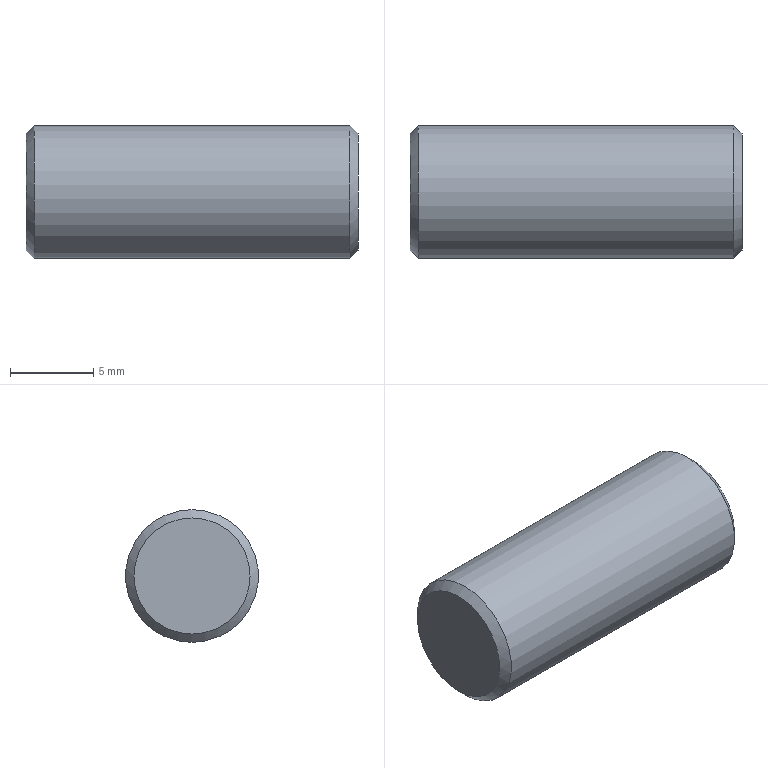Component | NX | DOWEL_PIN_8X20_2 | 1 solid | 5 faces | box 20 x 8 x 8 mm | volume 999 mm3 | plane 2 | cone 2 | cylinder 1 | commonest cylinder face diameters 8 x1
STEP:
#1=CARTESIAN_POINT('',(0.,0.,0.));
#2=DIRECTION('',(0.,0.,1.));
#3=DIRECTION('',(1.,0.,0.));
#4=AXIS2_PLACEMENT_3D('',#1,#2,#3);
#5=CARTESIAN_POINT('',(22.511,163.604,81.));
#6=VERTEX_POINT('',#5);
#7=CARTESIAN_POINT('',(22.511,163.604,85.));
#8=DIRECTION('',(-1.,0.,0.));
#9=DIRECTION('',(0.,0.,-1.));
#10=AXIS2_PLACEMENT_3D('',#7,#8,#9);
#11=CIRCLE('',#10,4.);
#12=CARTESIAN_POINT('',(23.011,163.604,85.));
#13=DIRECTION('',(-1.,0.,0.));
#14=DIRECTION('',(0.,0.,1.));
#15=AXIS2_PLACEMENT_3D('',#12,#13,#14);
#16=CYLINDRICAL_SURFACE('',#15,4.);
#17=CARTESIAN_POINT('',(3.142,0.5));
#18=DIRECTION('',(1.,0.));
#19=VECTOR('',#18,1.);
#20=LINE('',#17,#19);
#21=(GEOMETRIC_REPRESENTATION_CONTEXT(2)PARAMETRIC_REPRESENTATION_CONTEXT()REPRESENTATION_CONTEXT('',''));
#22=DEFINITIONAL_REPRESENTATION('',(#20),#21);
#23=PCURVE('',#16,#22);
#24=CARTESIAN_POINT('',(23.011,163.604,85.));
#25=DIRECTION('',(-1.,0.,0.));
#26=DIRECTION('',(0.,0.,1.));
#27=AXIS2_PLACEMENT_3D('',#24,#25,#26);
#28=CONICAL_SURFACE('',#27,3.5,0.7854);
#29=CARTESIAN_POINT('',(3.142,0.5));
#30=DIRECTION('',(1.,0.));
#31=VECTOR('',#30,1.);
#32=LINE('',#29,#31);
#33=(GEOMETRIC_REPRESENTATION_CONTEXT(2)PARAMETRIC_REPRESENTATION_CONTEXT()REPRESENTATION_CONTEXT('',''));
#34=DEFINITIONAL_REPRESENTATION('',(#32),#33);
#35=PCURVE('',#28,#34);
#36=SURFACE_CURVE('',#11,(#23,#35),.PCURVE_S1.);
#37=EDGE_CURVE('',#6,#6,#36,.T.);
#38=ORIENTED_EDGE('',*,*,#37,.T.);
#39=CARTESIAN_POINT('',(3.511,163.604,81.));
#40=VERTEX_POINT('',#39);
#41=CARTESIAN_POINT('',(22.511,163.604,81.));
#42=CARTESIAN_POINT('',(3.511,163.604,81.));
#43=B_SPLINE_CURVE_WITH_KNOTS('',1,(#41,#42),.UNSPECIFIED.,.F.,.F.,(2,2),(0.5,19.5),.PIECEWISE_BEZIER_KNOTS.);
#44=CARTESIAN_POINT('',(9.425,0.));
#45=DIRECTION('',(0.,1.));
#46=VECTOR('',#45,1.);
#47=LINE('',#44,#46);
#48=(GEOMETRIC_REPRESENTATION_CONTEXT(2)PARAMETRIC_REPRESENTATION_CONTEXT()REPRESENTATION_CONTEXT('',''));
#49=DEFINITIONAL_REPRESENTATION('',(#47),#48);
#50=PCURVE('',#16,#49);
#51=CARTESIAN_POINT('',(3.142,0.));
#52=DIRECTION('',(0.,1.));
#53=VECTOR('',#52,1.);
#54=LINE('',#51,#53);
#55=(GEOMETRIC_REPRESENTATION_CONTEXT(2)PARAMETRIC_REPRESENTATION_CONTEXT()REPRESENTATION_CONTEXT('',''));
#56=DEFINITIONAL_REPRESENTATION('',(#54),#55);
#57=PCURVE('',#16,#56);
#58=SEAM_CURVE('',#43,(#50,#57),.PCURVE_S1.);
#59=EDGE_CURVE('',#6,#40,#58,.T.);
#60=ORIENTED_EDGE('',*,*,#59,.T.);
#61=CARTESIAN_POINT('',(3.511,163.604,85.));
#62=DIRECTION('',(1.,0.,0.));
#63=DIRECTION('',(0.,0.,-1.));
#64=AXIS2_PLACEMENT_3D('',#61,#62,#63);
#65=CIRCLE('',#64,4.);
#66=CARTESIAN_POINT('',(9.425,19.5));
#67=DIRECTION('',(-1.,0.));
#68=VECTOR('',#67,1.);
#69=LINE('',#66,#68);
#70=(GEOMETRIC_REPRESENTATION_CONTEXT(2)PARAMETRIC_REPRESENTATION_CONTEXT()REPRESENTATION_CONTEXT('',''));
#71=DEFINITIONAL_REPRESENTATION('',(#69),#70);
#72=PCURVE('',#16,#71);
#73=CARTESIAN_POINT('',(3.511,163.604,85.));
#74=DIRECTION('',(1.,0.,0.));
#75=DIRECTION('',(0.,0.,-1.));
#76=AXIS2_PLACEMENT_3D('',#73,#74,#75);
#77=CONICAL_SURFACE('',#76,4.,0.7854);
#78=CARTESIAN_POINT('',(0.,0.));
#79=DIRECTION('',(1.,0.));
#80=VECTOR('',#79,1.);
#81=LINE('',#78,#80);
#82=(GEOMETRIC_REPRESENTATION_CONTEXT(2)PARAMETRIC_REPRESENTATION_CONTEXT()REPRESENTATION_CONTEXT('',''));
#83=DEFINITIONAL_REPRESENTATION('',(#81),#82);
#84=PCURVE('',#77,#83);
#85=SURFACE_CURVE('',#65,(#72,#84),.PCURVE_S1.);
#86=EDGE_CURVE('',#40,#40,#85,.T.);
#87=ORIENTED_EDGE('',*,*,#86,.T.);
#88=ORIENTED_EDGE('',*,*,#59,.F.);
#89=EDGE_LOOP('',(#38,#60,#87,#88));
#90=FACE_BOUND('',#89,.T.);
#91=ADVANCED_FACE('',(#90),#16,.T.);
#92=CARTESIAN_POINT('',(23.011,163.604,81.5));
#93=VERTEX_POINT('',#92);
#94=CARTESIAN_POINT('',(23.011,163.604,85.));
#95=DIRECTION('',(1.,0.,0.));
#96=DIRECTION('',(0.,0.,-1.));
#97=AXIS2_PLACEMENT_3D('',#94,#95,#96);
#98=CIRCLE('',#97,3.5);
#99=CARTESIAN_POINT('',(23.011,163.604,85.));
#100=DIRECTION('',(1.,0.,0.));
#101=DIRECTION('',(0.,0.,-1.));
#102=AXIS2_PLACEMENT_3D('',#99,#100,#101);
#103=PLANE('',#102);
#104=CARTESIAN_POINT('',(0.,0.));
#105=DIRECTION('',(1.,0.));
#106=AXIS2_PLACEMENT_2D('',#104,#105);
#107=CIRCLE('',#106,3.5);
#108=(GEOMETRIC_REPRESENTATION_CONTEXT(2)PARAMETRIC_REPRESENTATION_CONTEXT()REPRESENTATION_CONTEXT('',''));
#109=DEFINITIONAL_REPRESENTATION('',(#107),#108);
#110=PCURVE('',#103,#109);
#111=CARTESIAN_POINT('',(9.425,0.));
#112=DIRECTION('',(-1.,0.));
#113=VECTOR('',#112,1.);
#114=LINE('',#111,#113);
#115=(GEOMETRIC_REPRESENTATION_CONTEXT(2)PARAMETRIC_REPRESENTATION_CONTEXT()REPRESENTATION_CONTEXT('',''));
#116=DEFINITIONAL_REPRESENTATION('',(#114),#115);
#117=PCURVE('',#28,#116);
#118=SURFACE_CURVE('',#98,(#110,#117),.PCURVE_S1.);
#119=EDGE_CURVE('',#93,#93,#118,.T.);
#120=ORIENTED_EDGE('',*,*,#119,.T.);
#121=EDGE_LOOP('',(#120));
#122=FACE_BOUND('',#121,.T.);
#123=ADVANCED_FACE('',(#122),#103,.T.);
#124=CARTESIAN_POINT('',(3.011,163.604,81.5));
#125=VERTEX_POINT('',#124);
#126=CARTESIAN_POINT('',(3.011,163.604,85.));
#127=DIRECTION('',(-1.,0.,0.));
#128=DIRECTION('',(0.,0.,-1.));
#129=AXIS2_PLACEMENT_3D('',#126,#127,#128);
#130=CIRCLE('',#129,3.5);
#131=CARTESIAN_POINT('',(3.011,163.604,85.));
#132=DIRECTION('',(1.,0.,0.));
#133=DIRECTION('',(0.,0.,-1.));
#134=AXIS2_PLACEMENT_3D('',#131,#132,#133);
#135=PLANE('',#134);
#136=CARTESIAN_POINT('',(3.5,0.));
#137=CARTESIAN_POINT('',(3.5,-6.062));
#138=CARTESIAN_POINT('',(-1.75,-3.031));
#139=CARTESIAN_POINT('',(-7.,-0.));
#140=CARTESIAN_POINT('',(-1.75,3.031));
#141=CARTESIAN_POINT('',(3.5,6.062));
#142=CARTESIAN_POINT('',(3.5,0.));
#143=(BOUNDED_CURVE()B_SPLINE_CURVE(2,(#136,#137,#138,#139,#140,#141,#142),.UNSPECIFIED.,.T.,.F.)B_SPLINE_CURVE_WITH_KNOTS((1,2,2,2,2,1),(-2.094,0.,2.094,4.189,6.283,8.378),.UNSPECIFIED.)CURVE()GEOMETRIC_REPRESENTATION_ITEM()RATIONAL_B_SPLINE_CURVE((1.,0.5,1.,0.5,1.,0.5,1.))REPRESENTATION_ITEM(''));
#144=(GEOMETRIC_REPRESENTATION_CONTEXT(2)PARAMETRIC_REPRESENTATION_CONTEXT()REPRESENTATION_CONTEXT('',''));
#145=DEFINITIONAL_REPRESENTATION('',(#143),#144);
#146=PCURVE('',#135,#145);
#147=CARTESIAN_POINT('',(6.283,-0.5));
#148=DIRECTION('',(-1.,0.));
#149=VECTOR('',#148,1.);
#150=LINE('',#147,#149);
#151=(GEOMETRIC_REPRESENTATION_CONTEXT(2)PARAMETRIC_REPRESENTATION_CONTEXT()REPRESENTATION_CONTEXT('',''));
#152=DEFINITIONAL_REPRESENTATION('',(#150),#151);
#153=PCURVE('',#77,#152);
#154=SURFACE_CURVE('',#130,(#146,#153),.PCURVE_S1.);
#155=EDGE_CURVE('',#125,#125,#154,.T.);
#156=ORIENTED_EDGE('',*,*,#155,.T.);
#157=EDGE_LOOP('',(#156));
#158=FACE_BOUND('',#157,.T.);
#159=ADVANCED_FACE('',(#158),#135,.F.);
#160=ORIENTED_EDGE('',*,*,#37,.F.);
#161=CARTESIAN_POINT('',(23.011,163.604,81.5));
#162=CARTESIAN_POINT('',(22.511,163.604,81.));
#163=B_SPLINE_CURVE_WITH_KNOTS('',1,(#161,#162),.UNSPECIFIED.,.F.,.F.,(2,2),(0.,0.7071),.PIECEWISE_BEZIER_KNOTS.);
#164=CARTESIAN_POINT('',(3.142,0.));
#165=DIRECTION('',(0.,1.));
#166=VECTOR('',#165,1.);
#167=LINE('',#164,#166);
#168=(GEOMETRIC_REPRESENTATION_CONTEXT(2)PARAMETRIC_REPRESENTATION_CONTEXT()REPRESENTATION_CONTEXT('',''));
#169=DEFINITIONAL_REPRESENTATION('',(#167),#168);
#170=PCURVE('',#28,#169);
#171=CARTESIAN_POINT('',(9.425,0.));
#172=DIRECTION('',(0.,1.));
#173=VECTOR('',#172,1.);
#174=LINE('',#171,#173);
#175=(GEOMETRIC_REPRESENTATION_CONTEXT(2)PARAMETRIC_REPRESENTATION_CONTEXT()REPRESENTATION_CONTEXT('',''));
#176=DEFINITIONAL_REPRESENTATION('',(#174),#175);
#177=PCURVE('',#28,#176);
#178=SEAM_CURVE('',#163,(#170,#177),.PCURVE_S1.);
#179=EDGE_CURVE('',#93,#6,#178,.T.);
#180=ORIENTED_EDGE('',*,*,#179,.F.);
#181=ORIENTED_EDGE('',*,*,#119,.F.);
#182=ORIENTED_EDGE('',*,*,#179,.T.);
#183=EDGE_LOOP('',(#160,#180,#181,#182));
#184=FACE_BOUND('',#183,.T.);
#185=ADVANCED_FACE('',(#184),#28,.T.);
#186=ORIENTED_EDGE('',*,*,#155,.F.);
#187=CARTESIAN_POINT('',(3.011,163.604,81.5));
#188=CARTESIAN_POINT('',(3.511,163.604,81.));
#189=B_SPLINE_CURVE_WITH_KNOTS('',1,(#187,#188),.UNSPECIFIED.,.F.,.F.,(2,2),(-0.7071,0.),.PIECEWISE_BEZIER_KNOTS.);
#190=CARTESIAN_POINT('',(6.283,0.));
#191=DIRECTION('',(0.,1.));
#192=VECTOR('',#191,1.);
#193=LINE('',#190,#192);
#194=(GEOMETRIC_REPRESENTATION_CONTEXT(2)PARAMETRIC_REPRESENTATION_CONTEXT()REPRESENTATION_CONTEXT('',''));
#195=DEFINITIONAL_REPRESENTATION('',(#193),#194);
#196=PCURVE('',#77,#195);
#197=CARTESIAN_POINT('',(0.,0.));
#198=DIRECTION('',(0.,1.));
#199=VECTOR('',#198,1.);
#200=LINE('',#197,#199);
#201=(GEOMETRIC_REPRESENTATION_CONTEXT(2)PARAMETRIC_REPRESENTATION_CONTEXT()REPRESENTATION_CONTEXT('',''));
#202=DEFINITIONAL_REPRESENTATION('',(#200),#201);
#203=PCURVE('',#77,#202);
#204=SEAM_CURVE('',#189,(#196,#203),.PCURVE_S1.);
#205=EDGE_CURVE('',#125,#40,#204,.T.);
#206=ORIENTED_EDGE('',*,*,#205,.T.);
#207=ORIENTED_EDGE('',*,*,#86,.F.);
#208=ORIENTED_EDGE('',*,*,#205,.F.);
#209=EDGE_LOOP('',(#186,#206,#207,#208));
#210=FACE_BOUND('',#209,.T.);
#211=ADVANCED_FACE('',(#210),#77,.T.);
#212=CLOSED_SHELL('',(#91,#123,#159,#185,#211));
#213=MANIFOLD_SOLID_BREP('',#212);
#214=(LENGTH_UNIT()NAMED_UNIT(*)SI_UNIT(.MILLI.,.METRE.));
#215=UNCERTAINTY_MEASURE_WITH_UNIT(LENGTH_MEASURE(0.00001),#214,'','');
#216=(NAMED_UNIT(*)PLANE_ANGLE_UNIT()SI_UNIT($,.RADIAN.));
#217=(NAMED_UNIT(*)SI_UNIT($,.STERADIAN.)SOLID_ANGLE_UNIT());
#218=(GEOMETRIC_REPRESENTATION_CONTEXT(3)GLOBAL_UNCERTAINTY_ASSIGNED_CONTEXT((#215))GLOBAL_UNIT_ASSIGNED_CONTEXT((#214,#216,#217))REPRESENTATION_CONTEXT('',''));
#219=ADVANCED_BREP_SHAPE_REPRESENTATION('',(#4,#213),#218);